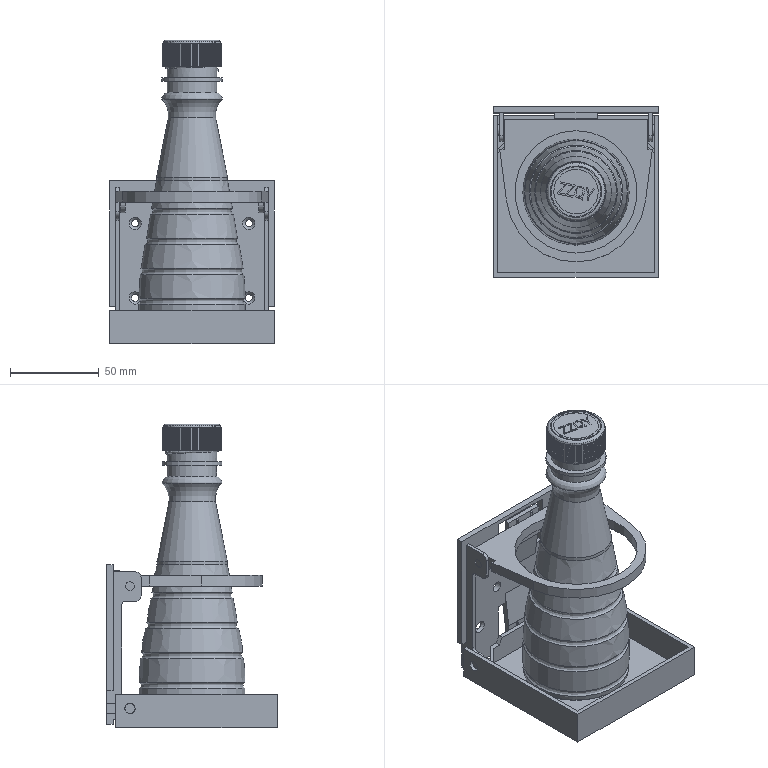Assembly | NX | mm | 5 component files | 5 solids | 519 faces | box 93 x 96 x 171.35 mm | volume 92363 mm3 | plane 232 | cylinder 222 | torus 24 | other 19 | spline 13 | cone 9 | commonest cylinder face diameters 33 x80 0.6 x80 6 x11 9 x10 4 x8 28 x5 12 x4 5 x4
Bill of materials:
unnamed part 1 | 1 |  | Shallow, roughly square open tray: a flat floor with low perimeter walls. Two opposite side walls rise into taller end portions, and each has a through-hole near its end. One wall has a stepped, notched top profile.
unnamed part 2 | 1 |  | Flat plate with a large circular through-opening. The outline is rounded on one end and has a straight, wider edge on the other, with angled sides between them. Short cylindrical pins stick out sideways from both ends of the straight edge, at a rounded knuckle-like boss. There is a small block under the middle of the straight edge.
unnamed part 3 | 1 |  | Short cylindrical cap-like part. The side wall has fine vertical knurling or ribbing, the top edge is rounded, and the top face is flat with a recessed circular line and letter-like characters engraved or embossed on it.
unnamed part 4 | 1 |  | Flat rectangular mounting plate with flanges along two opposite edges. Each flange ends in a rounded lug with a hole at one end and a rounded lug with a sideways pin at the other. The plate has four corner holes with chamfered or countersunk edges, a row of three central holes (the middle one larger and chamfered), and two rectangular windows containing tongue-like tab features.
unnamed part 5 | 1 |  | Bottle-shaped hollow body of revolution. It has an open neck with external helical thread-like ridges and a protruding neck ring flange, a short shoulder, a tapered body widening toward the base, several circumferential ribs or grooves around the lower body, and a flat base.
Mates:
1. fix | ZDBZZJ_02_Base 1 component
2. touch align | ZDBZZJ_01_Bracket 1 face | ZDBZZJ_02_Base 1 face
3. touch align | ZDBZZJ_01_Bracket 1 face | ZDBZZJ_02_Base 1 face
4. touch align | ZDBZZJ_03_Retainer 1 face | ZDBZZJ_01_Bracket 1 face
5. touch align | ZDBZZJ_03_Retainer 1 edge | ZDBZZJ_01_Bracket 1 face
6. touch align | BeverageBottle 1 face | ZDBZZJ_03_Retainer 1 face
7. touch align | BeverageBottle 1 face | ZDBZZJ_02_Base 1 face
8. touch align | ZDBZZ_05_BottleCap 1 face | BeverageBottle 1 face
9. touch align | ZDBZZ_05_BottleCap 1 face | BeverageBottle 1 face